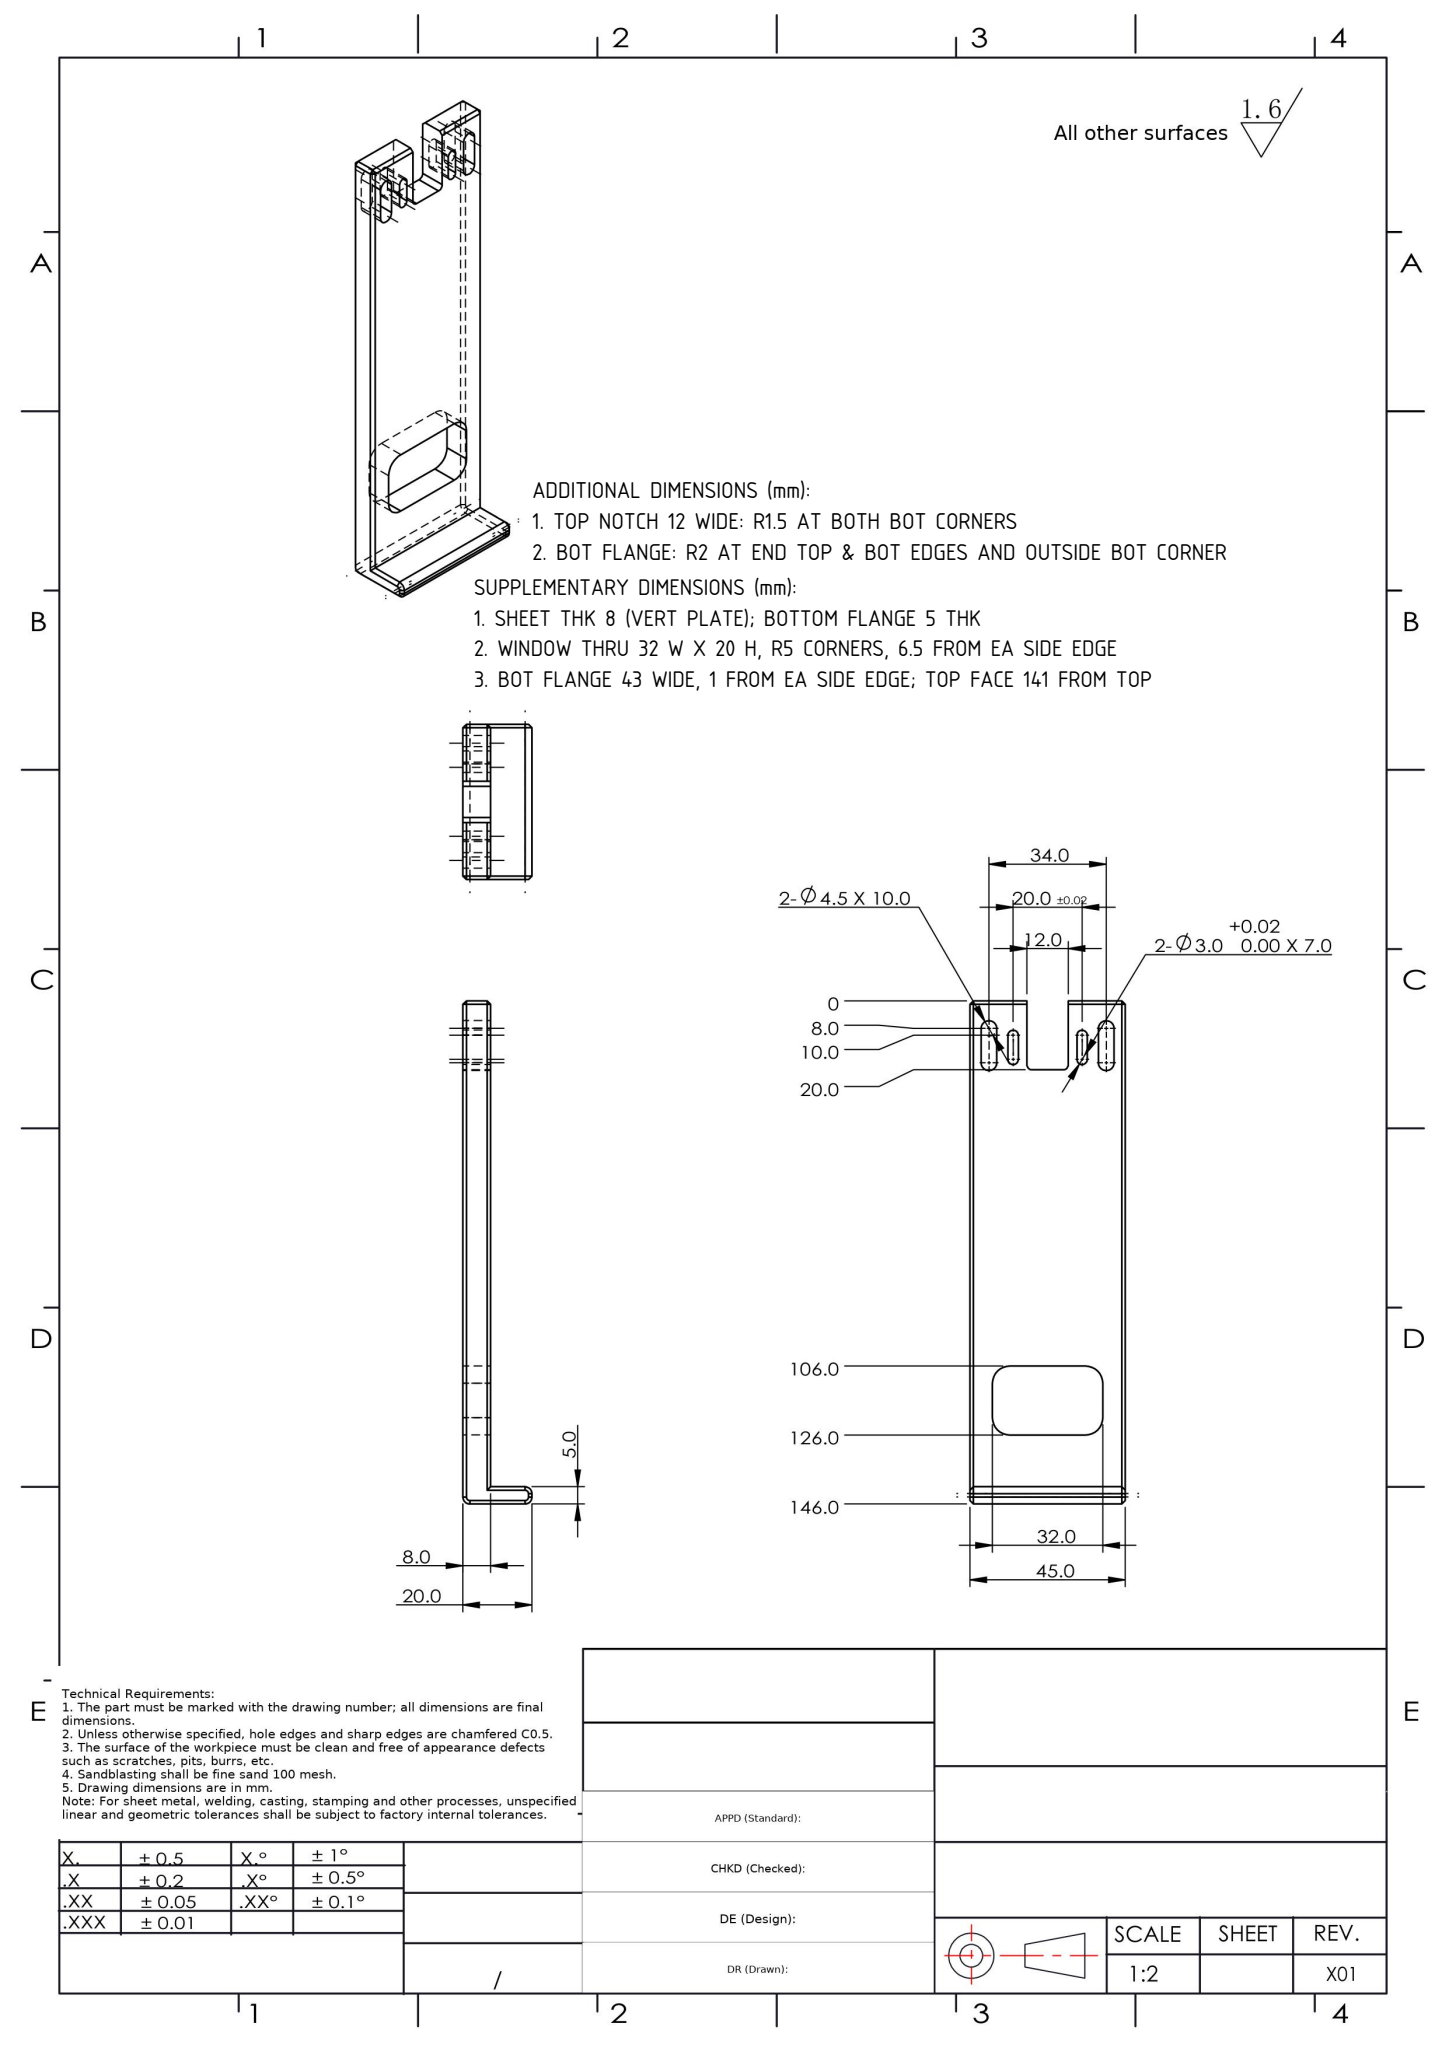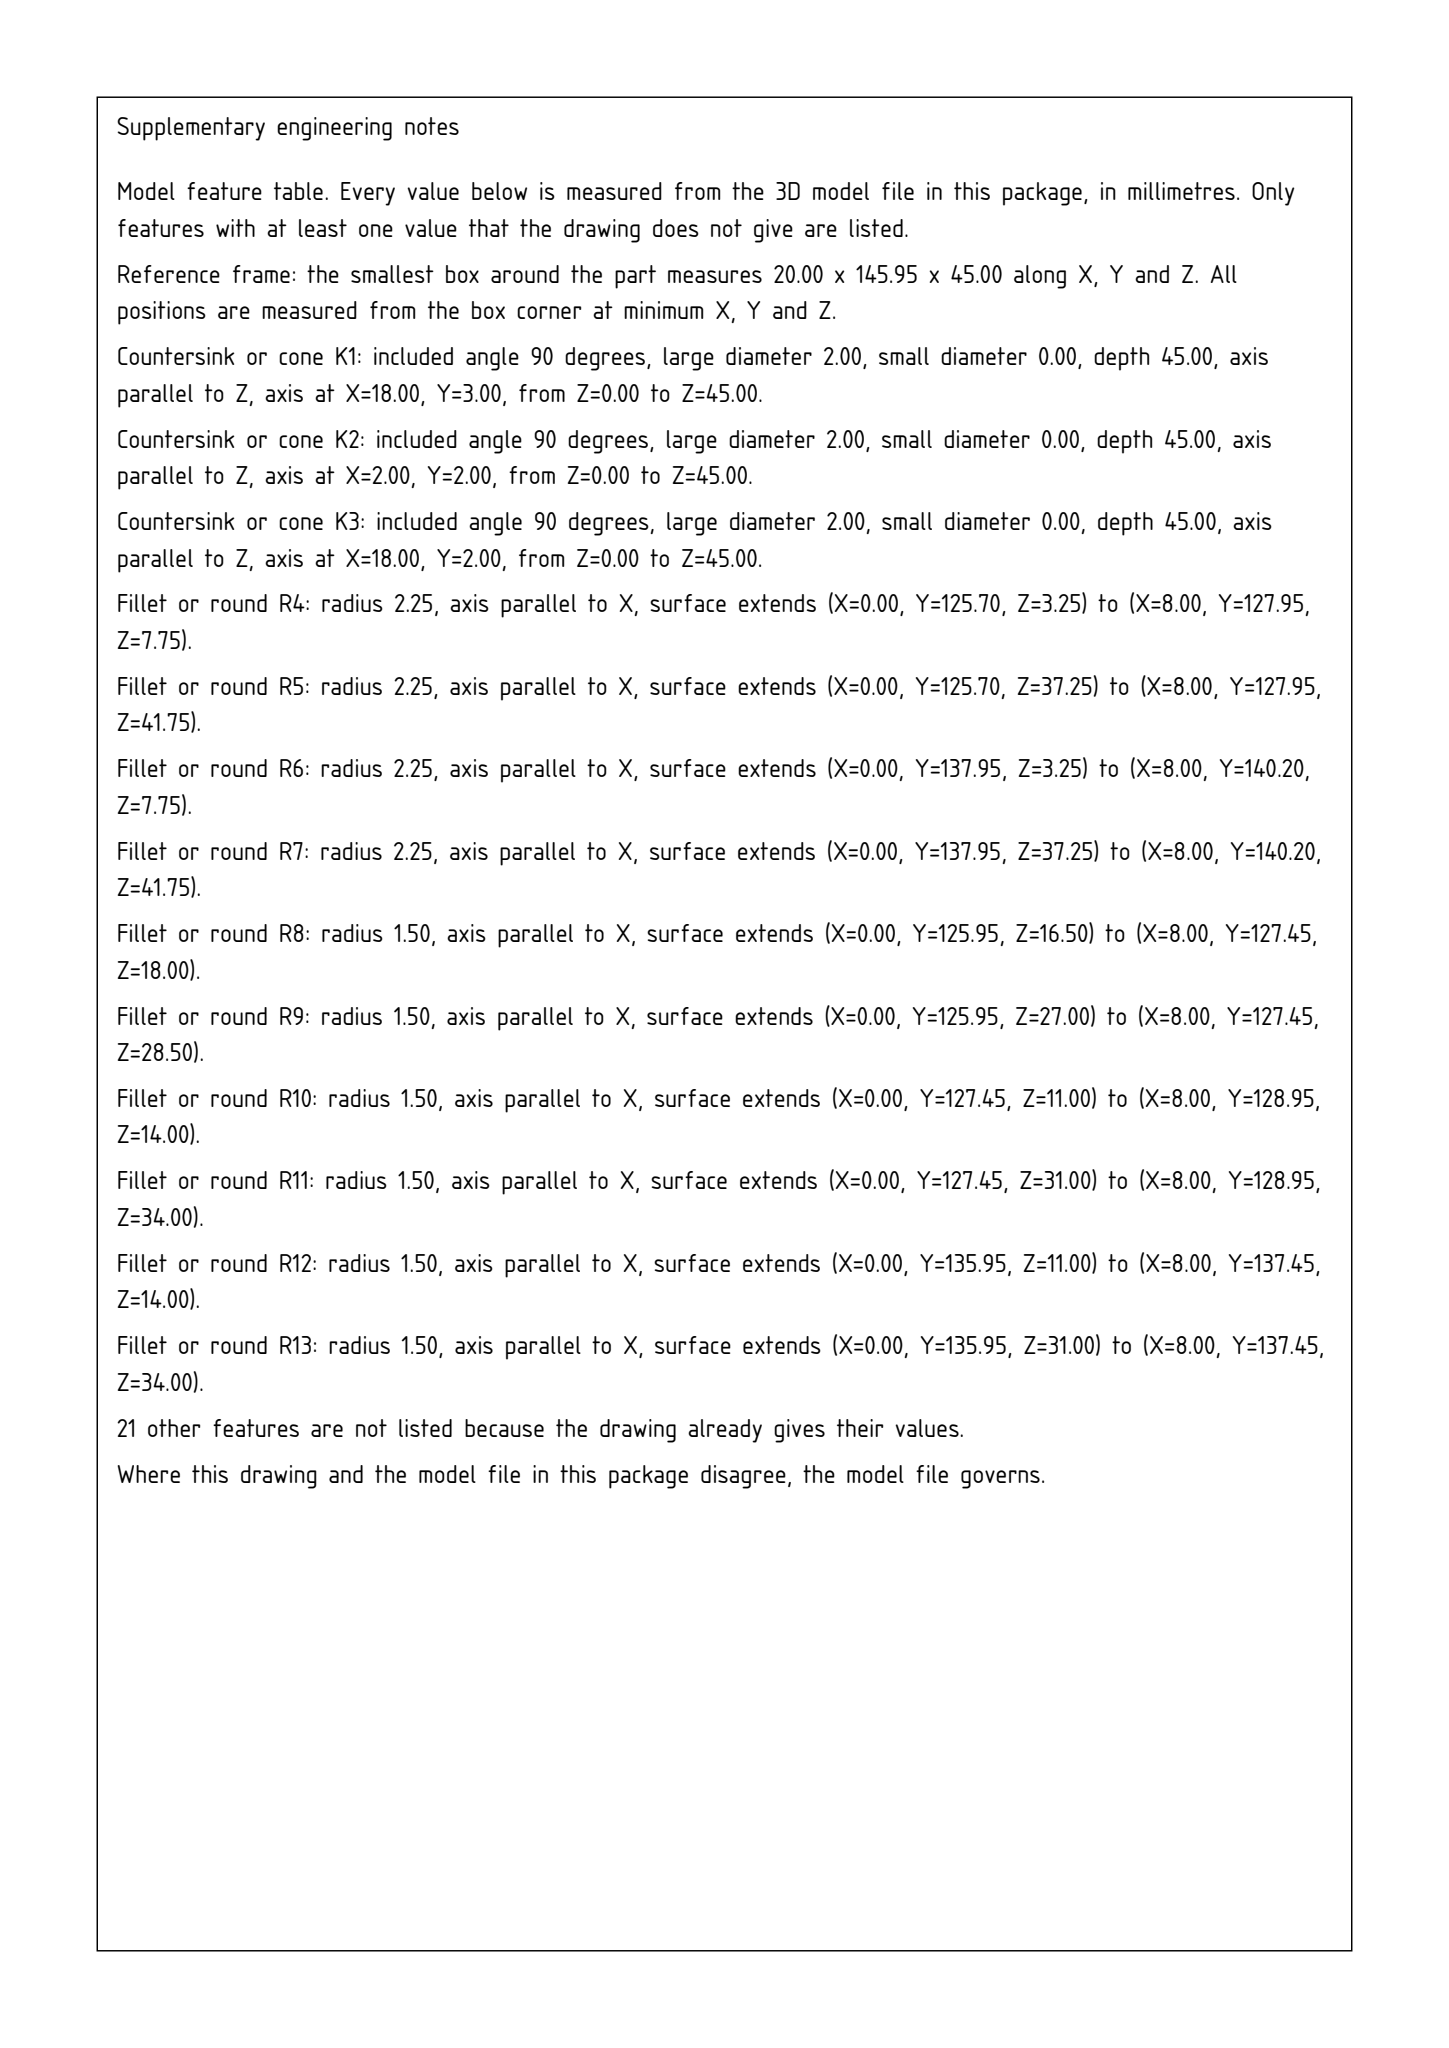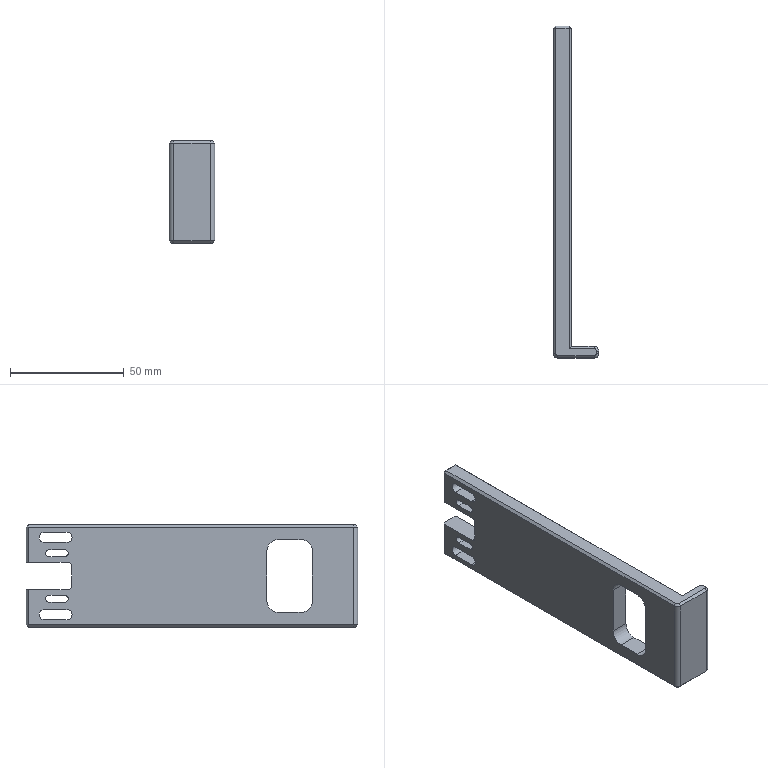Part | SolidWorks | mm | 1 solid | 71 faces | box 20 x 145.95 x 45 mm | volume 46483 mm3 | plane 44 | cylinder 21 | cone 6 | commonest cylinder face diameters 3 x8 4.5 x6 10 x4 4 x3
build123d program:
from build123d import *

# Parameters (mm, degrees)
SKETCH1_W           = 8
SKETCH1_H           = 145.95
SKETCH1_W_2         = 12
SKETCH1_H_2         = 5
BOSS_EXTRUDE1_DEPTH = 45
CUT_EXTRUDE1_DEPTH  = 60
CUT_EXTRUDE2_DEPTH  = 4
SKETCH4_W           = 12
SKETCH4_H           = 20
CUT_EXTRUDE3_DEPTH  = 155.034
SKETCH5_W           = 32
SKETCH5_H           = 20
CUT_EXTRUDE4_DEPTH  = 155.034
FILLET1_R           = 2
CHAMFER1_SIZE       = 1
FILLET2_R           = 5
FILLET3_R           = 1.5
BOSS_EXTRUDE3_DEPTH = 4


with BuildPart() as part:
    # Sketch1 → Boss-Extrude1 (new body)
    with BuildSketch(Plane.XY):
        with Locations((4, -72.975)):
            Rectangle(SKETCH1_W, SKETCH1_H)
        with Locations((14, -143.45)):
            Rectangle(SKETCH1_W_2, SKETCH1_H_2)
    extrude(amount=BOSS_EXTRUDE1_DEPTH)

    # Sketch2 → Cut-Extrude1 (cut)
    with BuildSketch(Plane.ZY):
        with BuildLine():
            Line((7.75, -8), (7.75, -18))
            ThreePointArc((7.75, -18), (5.5, -20.25), (3.25, -18))
            Line((3.25, -18), (3.25, -8))
            ThreePointArc((3.25, -8), (5.5, -5.75), (7.75, -8))
        make_face()
        with BuildLine():
            Line((41.75, -8), (41.75, -18))
            ThreePointArc((41.75, -18), (39.5, -20.25), (37.25, -18))
            Line((37.25, -18), (37.25, -8))
            ThreePointArc((37.25, -8), (39.5, -5.75), (41.75, -8))
        make_face()
        with BuildLine():
            Line((14, -10), (14, -17))
            ThreePointArc((14, -17), (12.5, -18.5), (11, -17))
            Line((11, -17), (11, -10))
            ThreePointArc((11, -10), (12.5, -8.5), (14, -10))
        make_face()
        with BuildLine():
            Line((34, -10), (34, -17))
            ThreePointArc((34, -17), (32.5, -18.5), (31, -17))
            Line((31, -17), (31, -10))
            ThreePointArc((31, -10), (32.5, -8.5), (34, -10))
        make_face()
    extrude(amount=-CUT_EXTRUDE1_DEPTH, mode=Mode.SUBTRACT)

    # Sketch3 → Cut-Extrude2 (cut)
    with BuildSketch(Plane.ZY):
        with BuildLine():
            Line((9.5, -8), (9.5, -18))
            ThreePointArc((9.5, -18), (5.5, -22), (1.5, -18))
            Line((1.5, -18), (1.5, -8))
            ThreePointArc((1.5, -8), (5.5, -4), (9.5, -8))
        make_face()
        with BuildLine():
            Line((43.5, -8), (43.5, -18))
            ThreePointArc((43.5, -18), (39.5, -22), (35.5, -18))
            Line((35.5, -18), (35.5, -8))
            ThreePointArc((35.5, -8), (39.5, -4), (43.5, -8))
        make_face()
    extrude(amount=-CUT_EXTRUDE2_DEPTH, mode=Mode.SUBTRACT)

    # Sketch4 → Cut-Extrude3 (cut, through all)
    with BuildSketch(Plane.ZY):
        with Locations((22.5, -10)):
            Rectangle(SKETCH4_W, SKETCH4_H)
    extrude(amount=-CUT_EXTRUDE3_DEPTH, mode=Mode.SUBTRACT)

    # Sketch5 → Cut-Extrude4 (cut, through all)
    with BuildSketch(Plane.ZY):
        with Locations((22.5, -115.95)):
            Rectangle(SKETCH5_W, SKETCH5_H)
    extrude(amount=-CUT_EXTRUDE4_DEPTH, mode=Mode.SUBTRACT)

    # Fillet1
    fillet1_edges = [part.edges().sort_by_distance(p)[0] for p in [
        (20, -140.95, 22.5),
        (20, -145.95, 22.5),
        (0, -145.95, 22.5),
    ]]
    fillet(fillet1_edges, radius=FILLET1_R)

    # Chamfer1
    chamfer1_edges = [part.edges().sort_by_distance(p)[0] for p in [
        (0, 0, 36.75),
        (8, 0, 36.75),
        (0, -71.975, 45),
        (0, 0, 8.25),
        (8, 0, 8.25),
        (10, -145.95, 0),
        (10, -145.95, 45),
        (20, -143.45, 0),
        (19.414, -141.536, 0),
        (19.414, -145.364, 0),
        (0.5858, -145.364, 0),
        (20, -143.45, 45),
        (19.414, -141.536, 45),
        (19.414, -145.364, 45),
        (0.5858, -145.364, 45),
        (13, -140.95, 45),
        (8, -70.475, 45),
        (13, -140.95, 0),
        (0, -71.975, 0),
        (4, 0, 45),
        (4, 0, 0),
        (8, -70.475, 0),
    ]]
    chamfer(chamfer1_edges, length=CHAMFER1_SIZE)

    # Fillet2
    fillet2_edges = [part.edges().sort_by_distance(p)[0] for p in [
        (4, -125.95, 6.5),
        (4, -105.95, 6.5),
        (4, -105.95, 38.5),
        (4, -125.95, 38.5),
    ]]
    fillet(fillet2_edges, radius=FILLET2_R)

    # Fillet3
    fillet3_edges = [part.edges().sort_by_distance(p)[0] for p in [
        (4, -20, 16.5),
        (4, -20, 28.5),
    ]]
    fillet(fillet3_edges, radius=FILLET3_R)

    # Sketch7 → Boss-Extrude3 (add)
    # profile 1 of 2: a face of its own
    with BuildSketch(Plane.ZY):
        with BuildLine():
            Line((1.5, -8), (1.5, -18))
            ThreePointArc((1.5, -18), (5.5, -22), (9.5, -18))
            Line((9.5, -18), (9.5, -8))
            ThreePointArc((9.5, -8), (5.5, -4), (1.5, -8))
        make_face()
        with BuildLine():
            Line((3.25, -18), (3.25, -8))
            ThreePointArc((3.25, -8), (5.5, -5.75), (7.75, -8))
            Line((7.75, -8), (7.75, -18))
            ThreePointArc((7.75, -18), (5.5, -20.25), (3.25, -18))
        make_face(mode=Mode.SUBTRACT)
    # profile 2 of 2: a face of its own
    with BuildSketch(Plane.ZY):
        with BuildLine():
            Line((35.5, -8), (35.5, -18))
            ThreePointArc((35.5, -18), (39.5, -22), (43.5, -18))
            Line((43.5, -18), (43.5, -8))
            ThreePointArc((43.5, -8), (39.5, -4), (35.5, -8))
        make_face()
        with BuildLine():
            Line((37.25, -18), (37.25, -8))
            ThreePointArc((37.25, -8), (39.5, -5.75), (41.75, -8))
            Line((41.75, -8), (41.75, -18))
            ThreePointArc((41.75, -18), (39.5, -20.25), (37.25, -18))
        make_face(mode=Mode.SUBTRACT)
    extrude(amount=-BOSS_EXTRUDE3_DEPTH)


solid = part.part